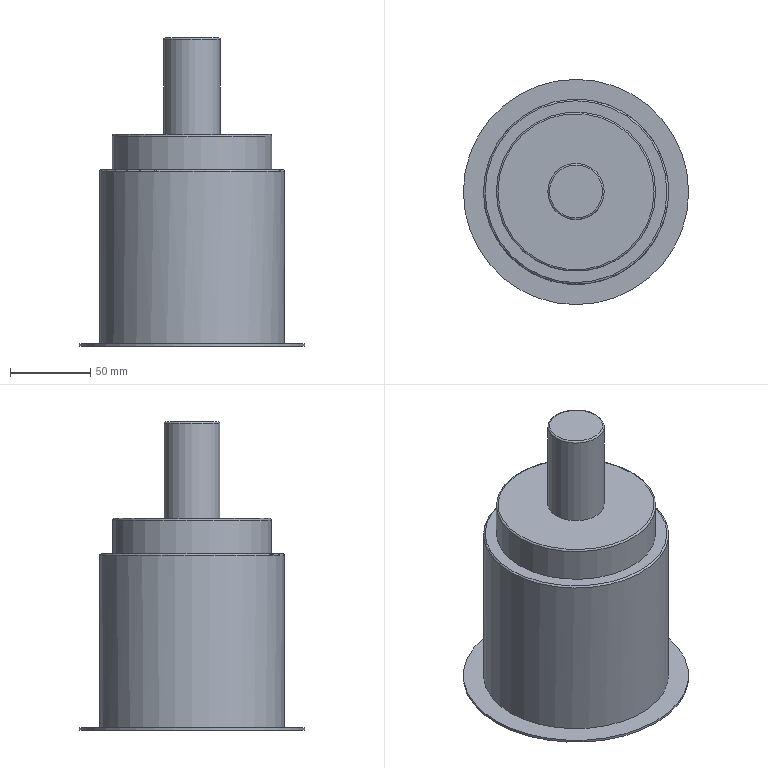Component | NX | A_PART_6 | 1 solid | 12 faces | box 140 x 140 x 191.5 mm | volume 1371784 mm3 | plane 5 | cylinder 4 | torus 3 | commonest cylinder face diameters 99 x1 35 x1 115 x1 140 x1
STEP:
#1=CARTESIAN_POINT('',(0.,0.,0.));
#2=DIRECTION('',(0.,0.,1.));
#3=DIRECTION('',(1.,0.,0.));
#4=AXIS2_PLACEMENT_3D('',#1,#2,#3);
#5=CARTESIAN_POINT('',(303.417,257.136,29.984));
#6=VERTEX_POINT('',#5);
#7=CARTESIAN_POINT('',(352.917,257.26,29.984));
#8=DIRECTION('',(0.,0.,-1.));
#9=DIRECTION('',(-1.,-0.0025,0.));
#10=AXIS2_PLACEMENT_3D('',#7,#8,#9);
#11=CIRCLE('',#10,49.5);
#12=CARTESIAN_POINT('',(352.917,257.26,30.984));
#13=DIRECTION('',(0.,0.,-1.));
#14=DIRECTION('',(-1.,-0.0025,0.));
#15=AXIS2_PLACEMENT_3D('',#12,#13,#14);
#16=CYLINDRICAL_SURFACE('',#15,49.5);
#17=CARTESIAN_POINT('',(0.,1.));
#18=DIRECTION('',(1.,0.));
#19=VECTOR('',#18,1.);
#20=LINE('',#17,#19);
#21=(GEOMETRIC_REPRESENTATION_CONTEXT(2)PARAMETRIC_REPRESENTATION_CONTEXT()REPRESENTATION_CONTEXT('',''));
#22=DEFINITIONAL_REPRESENTATION('',(#20),#21);
#23=PCURVE('',#16,#22);
#24=CARTESIAN_POINT('',(352.917,257.26,29.984));
#25=DIRECTION('',(0.,0.,-1.));
#26=DIRECTION('',(-1.,-0.0025,0.));
#27=AXIS2_PLACEMENT_3D('',#24,#25,#26);
#28=TOROIDAL_SURFACE('',#27,48.5,1.);
#29=CARTESIAN_POINT('',(0.,6.283));
#30=DIRECTION('',(1.,0.));
#31=VECTOR('',#30,1.);
#32=LINE('',#29,#31);
#33=(GEOMETRIC_REPRESENTATION_CONTEXT(2)PARAMETRIC_REPRESENTATION_CONTEXT()REPRESENTATION_CONTEXT('',''));
#34=DEFINITIONAL_REPRESENTATION('',(#32),#33);
#35=PCURVE('',#28,#34);
#36=SURFACE_CURVE('',#11,(#23,#35),.PCURVE_S1.);
#37=EDGE_CURVE('',#6,#6,#36,.T.);
#38=ORIENTED_EDGE('',*,*,#37,.T.);
#39=CARTESIAN_POINT('',(303.417,257.136,8.984));
#40=VERTEX_POINT('',#39);
#41=CARTESIAN_POINT('',(303.417,257.136,29.984));
#42=CARTESIAN_POINT('',(303.417,257.136,8.984));
#43=B_SPLINE_CURVE_WITH_KNOTS('',1,(#41,#42),.UNSPECIFIED.,.F.,.F.,(2,2),(1.,22.),.PIECEWISE_BEZIER_KNOTS.);
#44=CARTESIAN_POINT('',(6.283,0.));
#45=DIRECTION('',(0.,1.));
#46=VECTOR('',#45,1.);
#47=LINE('',#44,#46);
#48=(GEOMETRIC_REPRESENTATION_CONTEXT(2)PARAMETRIC_REPRESENTATION_CONTEXT()REPRESENTATION_CONTEXT('',''));
#49=DEFINITIONAL_REPRESENTATION('',(#47),#48);
#50=PCURVE('',#16,#49);
#51=CARTESIAN_POINT('',(0.,0.));
#52=DIRECTION('',(0.,1.));
#53=VECTOR('',#52,1.);
#54=LINE('',#51,#53);
#55=(GEOMETRIC_REPRESENTATION_CONTEXT(2)PARAMETRIC_REPRESENTATION_CONTEXT()REPRESENTATION_CONTEXT('',''));
#56=DEFINITIONAL_REPRESENTATION('',(#54),#55);
#57=PCURVE('',#16,#56);
#58=SEAM_CURVE('',#43,(#50,#57),.PCURVE_S1.);
#59=EDGE_CURVE('',#6,#40,#58,.T.);
#60=ORIENTED_EDGE('',*,*,#59,.T.);
#61=CARTESIAN_POINT('',(352.917,257.26,8.984));
#62=DIRECTION('',(0.,0.,1.));
#63=DIRECTION('',(-1.,-0.0025,0.));
#64=AXIS2_PLACEMENT_3D('',#61,#62,#63);
#65=CIRCLE('',#64,49.5);
#66=CARTESIAN_POINT('',(6.283,22.));
#67=DIRECTION('',(-1.,0.));
#68=VECTOR('',#67,1.);
#69=LINE('',#66,#68);
#70=(GEOMETRIC_REPRESENTATION_CONTEXT(2)PARAMETRIC_REPRESENTATION_CONTEXT()REPRESENTATION_CONTEXT('',''));
#71=DEFINITIONAL_REPRESENTATION('',(#69),#70);
#72=PCURVE('',#16,#71);
#73=CARTESIAN_POINT('',(352.917,257.26,8.984));
#74=DIRECTION('',(0.,0.,-1.));
#75=DIRECTION('',(-1.,-0.0025,0.));
#76=AXIS2_PLACEMENT_3D('',#73,#74,#75);
#77=PLANE('',#76);
#78=CARTESIAN_POINT('',(49.5,-0.));
#79=CARTESIAN_POINT('',(49.5,-85.737));
#80=CARTESIAN_POINT('',(-24.75,-42.868));
#81=CARTESIAN_POINT('',(-99.,-0.));
#82=CARTESIAN_POINT('',(-24.75,42.868));
#83=CARTESIAN_POINT('',(49.5,85.737));
#84=CARTESIAN_POINT('',(49.5,-0.));
#85=(BOUNDED_CURVE()B_SPLINE_CURVE(2,(#78,#79,#80,#81,#82,#83,#84),.UNSPECIFIED.,.T.,.F.)B_SPLINE_CURVE_WITH_KNOTS((1,2,2,2,2,1),(-2.094,0.,2.094,4.189,6.283,8.378),.UNSPECIFIED.)CURVE()GEOMETRIC_REPRESENTATION_ITEM()RATIONAL_B_SPLINE_CURVE((1.,0.5,1.,0.5,1.,0.5,1.))REPRESENTATION_ITEM(''));
#86=(GEOMETRIC_REPRESENTATION_CONTEXT(2)PARAMETRIC_REPRESENTATION_CONTEXT()REPRESENTATION_CONTEXT('',''));
#87=DEFINITIONAL_REPRESENTATION('',(#85),#86);
#88=PCURVE('',#77,#87);
#89=SURFACE_CURVE('',#65,(#72,#88),.PCURVE_S1.);
#90=EDGE_CURVE('',#40,#40,#89,.T.);
#91=ORIENTED_EDGE('',*,*,#90,.T.);
#92=ORIENTED_EDGE('',*,*,#59,.F.);
#93=EDGE_LOOP('',(#38,#60,#91,#92));
#94=FACE_BOUND('',#93,.T.);
#95=ADVANCED_FACE('',(#94),#16,.T.);
#96=CARTESIAN_POINT('',(304.417,257.138,30.984));
#97=VERTEX_POINT('',#96);
#98=CARTESIAN_POINT('',(352.917,257.26,30.984));
#99=DIRECTION('',(0.,0.,1.));
#100=DIRECTION('',(-1.,-0.0025,0.));
#101=AXIS2_PLACEMENT_3D('',#98,#99,#100);
#102=CIRCLE('',#101,48.5);
#103=CARTESIAN_POINT('',(352.917,257.26,30.984));
#104=DIRECTION('',(0.,0.,-1.));
#105=DIRECTION('',(-1.,-0.0025,0.));
#106=AXIS2_PLACEMENT_3D('',#103,#104,#105);
#107=PLANE('',#106);
#108=CARTESIAN_POINT('',(48.5,-0.));
#109=CARTESIAN_POINT('',(48.5,-84.004));
#110=CARTESIAN_POINT('',(-24.25,-42.002));
#111=CARTESIAN_POINT('',(-97.,0.));
#112=CARTESIAN_POINT('',(-24.25,42.002));
#113=CARTESIAN_POINT('',(48.5,84.004));
#114=CARTESIAN_POINT('',(48.5,-0.));
#115=(BOUNDED_CURVE()B_SPLINE_CURVE(2,(#108,#109,#110,#111,#112,#113,#114),.UNSPECIFIED.,.T.,.F.)B_SPLINE_CURVE_WITH_KNOTS((1,2,2,2,2,1),(-2.094,0.,2.094,4.189,6.283,8.378),.UNSPECIFIED.)CURVE()GEOMETRIC_REPRESENTATION_ITEM()RATIONAL_B_SPLINE_CURVE((1.,0.5,1.,0.5,1.,0.5,1.))REPRESENTATION_ITEM(''));
#116=(GEOMETRIC_REPRESENTATION_CONTEXT(2)PARAMETRIC_REPRESENTATION_CONTEXT()REPRESENTATION_CONTEXT('',''));
#117=DEFINITIONAL_REPRESENTATION('',(#115),#116);
#118=PCURVE('',#107,#117);
#119=CARTESIAN_POINT('',(6.283,4.712));
#120=DIRECTION('',(-1.,0.));
#121=VECTOR('',#120,1.);
#122=LINE('',#119,#121);
#123=(GEOMETRIC_REPRESENTATION_CONTEXT(2)PARAMETRIC_REPRESENTATION_CONTEXT()REPRESENTATION_CONTEXT('',''));
#124=DEFINITIONAL_REPRESENTATION('',(#122),#123);
#125=PCURVE('',#28,#124);
#126=SURFACE_CURVE('',#102,(#118,#125),.PCURVE_S1.);
#127=EDGE_CURVE('',#97,#97,#126,.T.);
#128=ORIENTED_EDGE('',*,*,#127,.T.);
#129=EDGE_LOOP('',(#128));
#130=FACE_BOUND('',#129,.T.);
#131=CARTESIAN_POINT('',(370.417,257.303,30.984));
#132=VERTEX_POINT('',#131);
#133=CARTESIAN_POINT('',(335.417,257.216,30.984));
#134=VERTEX_POINT('',#133);
#135=CARTESIAN_POINT('',(352.917,257.26,30.984));
#136=DIRECTION('',(0.,0.,-1.));
#137=DIRECTION('',(1.,0.0025,0.));
#138=AXIS2_PLACEMENT_3D('',#135,#136,#137);
#139=CIRCLE('',#138,17.5);
#140=CARTESIAN_POINT('',(0.,0.));
#141=DIRECTION('',(-1.,0.));
#142=AXIS2_PLACEMENT_2D('',#140,#141);
#143=CIRCLE('',#142,17.5);
#144=(GEOMETRIC_REPRESENTATION_CONTEXT(2)PARAMETRIC_REPRESENTATION_CONTEXT()REPRESENTATION_CONTEXT('',''));
#145=DEFINITIONAL_REPRESENTATION('',(#143),#144);
#146=PCURVE('',#107,#145);
#147=CARTESIAN_POINT('',(352.917,257.26,90.984));
#148=DIRECTION('',(0.,0.,-1.));
#149=DIRECTION('',(-1.,-0.0025,0.));
#150=AXIS2_PLACEMENT_3D('',#147,#148,#149);
#151=CYLINDRICAL_SURFACE('',#150,17.5);
#152=CARTESIAN_POINT('',(3.142,60.));
#153=DIRECTION('',(1.,0.));
#154=VECTOR('',#153,1.);
#155=LINE('',#152,#154);
#156=(GEOMETRIC_REPRESENTATION_CONTEXT(2)PARAMETRIC_REPRESENTATION_CONTEXT()REPRESENTATION_CONTEXT('',''));
#157=DEFINITIONAL_REPRESENTATION('',(#155),#156);
#158=PCURVE('',#151,#157);
#159=SURFACE_CURVE('',#139,(#146,#158),.PCURVE_S1.);
#160=EDGE_CURVE('',#132,#134,#159,.T.);
#161=ORIENTED_EDGE('',*,*,#160,.T.);
#162=CARTESIAN_POINT('',(352.917,257.26,30.984));
#163=DIRECTION('',(0.,0.,-1.));
#164=DIRECTION('',(1.,0.0025,0.));
#165=AXIS2_PLACEMENT_3D('',#162,#163,#164);
#166=CIRCLE('',#165,17.5);
#167=CARTESIAN_POINT('',(0.,0.));
#168=DIRECTION('',(-1.,0.));
#169=AXIS2_PLACEMENT_2D('',#167,#168);
#170=CIRCLE('',#169,17.5);
#171=(GEOMETRIC_REPRESENTATION_CONTEXT(2)PARAMETRIC_REPRESENTATION_CONTEXT()REPRESENTATION_CONTEXT('',''));
#172=DEFINITIONAL_REPRESENTATION('',(#170),#171);
#173=PCURVE('',#107,#172);
#174=CARTESIAN_POINT('',(-3.142,60.));
#175=DIRECTION('',(1.,0.));
#176=VECTOR('',#175,1.);
#177=LINE('',#174,#176);
#178=(GEOMETRIC_REPRESENTATION_CONTEXT(2)PARAMETRIC_REPRESENTATION_CONTEXT()REPRESENTATION_CONTEXT('',''));
#179=DEFINITIONAL_REPRESENTATION('',(#177),#178);
#180=PCURVE('',#151,#179);
#181=SURFACE_CURVE('',#166,(#173,#180),.PCURVE_S1.);
#182=EDGE_CURVE('',#134,#132,#181,.T.);
#183=ORIENTED_EDGE('',*,*,#182,.T.);
#184=EDGE_LOOP('',(#161,#183));
#185=FACE_BOUND('',#184,.T.);
#186=ADVANCED_FACE('',(#130,#185),#107,.F.);
#187=CARTESIAN_POINT('',(335.417,257.216,89.984));
#188=VERTEX_POINT('',#187);
#189=CARTESIAN_POINT('',(352.917,257.26,89.984));
#190=DIRECTION('',(0.,0.,-1.));
#191=DIRECTION('',(-1.,-0.0025,0.));
#192=AXIS2_PLACEMENT_3D('',#189,#190,#191);
#193=CIRCLE('',#192,17.5);
#194=CARTESIAN_POINT('',(0.,1.));
#195=DIRECTION('',(1.,0.));
#196=VECTOR('',#195,1.);
#197=LINE('',#194,#196);
#198=(GEOMETRIC_REPRESENTATION_CONTEXT(2)PARAMETRIC_REPRESENTATION_CONTEXT()REPRESENTATION_CONTEXT('',''));
#199=DEFINITIONAL_REPRESENTATION('',(#197),#198);
#200=PCURVE('',#151,#199);
#201=CARTESIAN_POINT('',(352.917,257.26,89.984));
#202=DIRECTION('',(0.,0.,-1.));
#203=DIRECTION('',(-1.,-0.0025,0.));
#204=AXIS2_PLACEMENT_3D('',#201,#202,#203);
#205=TOROIDAL_SURFACE('',#204,16.5,1.);
#206=CARTESIAN_POINT('',(0.,6.283));
#207=DIRECTION('',(1.,0.));
#208=VECTOR('',#207,1.);
#209=LINE('',#206,#208);
#210=(GEOMETRIC_REPRESENTATION_CONTEXT(2)PARAMETRIC_REPRESENTATION_CONTEXT()REPRESENTATION_CONTEXT('',''));
#211=DEFINITIONAL_REPRESENTATION('',(#209),#210);
#212=PCURVE('',#205,#211);
#213=SURFACE_CURVE('',#193,(#200,#212),.PCURVE_S1.);
#214=EDGE_CURVE('',#188,#188,#213,.T.);
#215=ORIENTED_EDGE('',*,*,#214,.T.);
#216=CARTESIAN_POINT('',(335.417,257.216,89.984));
#217=CARTESIAN_POINT('',(335.417,257.216,30.984));
#218=B_SPLINE_CURVE_WITH_KNOTS('',1,(#216,#217),.UNSPECIFIED.,.F.,.F.,(2,2),(1.,60.),.PIECEWISE_BEZIER_KNOTS.);
#219=CARTESIAN_POINT('',(6.283,0.));
#220=DIRECTION('',(0.,1.));
#221=VECTOR('',#220,1.);
#222=LINE('',#219,#221);
#223=(GEOMETRIC_REPRESENTATION_CONTEXT(2)PARAMETRIC_REPRESENTATION_CONTEXT()REPRESENTATION_CONTEXT('',''));
#224=DEFINITIONAL_REPRESENTATION('',(#222),#223);
#225=PCURVE('',#151,#224);
#226=CARTESIAN_POINT('',(0.,0.));
#227=DIRECTION('',(0.,1.));
#228=VECTOR('',#227,1.);
#229=LINE('',#226,#228);
#230=(GEOMETRIC_REPRESENTATION_CONTEXT(2)PARAMETRIC_REPRESENTATION_CONTEXT()REPRESENTATION_CONTEXT('',''));
#231=DEFINITIONAL_REPRESENTATION('',(#229),#230);
#232=PCURVE('',#151,#231);
#233=SEAM_CURVE('',#218,(#225,#232),.PCURVE_S1.);
#234=EDGE_CURVE('',#188,#134,#233,.T.);
#235=ORIENTED_EDGE('',*,*,#234,.T.);
#236=ORIENTED_EDGE('',*,*,#160,.F.);
#237=ORIENTED_EDGE('',*,*,#182,.F.);
#238=ORIENTED_EDGE('',*,*,#234,.F.);
#239=EDGE_LOOP('',(#215,#235,#236,#237,#238));
#240=FACE_BOUND('',#239,.T.);
#241=ADVANCED_FACE('',(#240),#151,.T.);
#242=CARTESIAN_POINT('',(336.417,257.218,90.984));
#243=VERTEX_POINT('',#242);
#244=CARTESIAN_POINT('',(352.917,257.26,90.984));
#245=DIRECTION('',(0.,0.,1.));
#246=DIRECTION('',(-1.,-0.0025,0.));
#247=AXIS2_PLACEMENT_3D('',#244,#245,#246);
#248=CIRCLE('',#247,16.5);
#249=CARTESIAN_POINT('',(352.917,257.26,90.984));
#250=DIRECTION('',(0.,0.,-1.));
#251=DIRECTION('',(-1.,-0.0025,0.));
#252=AXIS2_PLACEMENT_3D('',#249,#250,#251);
#253=PLANE('',#252);
#254=CARTESIAN_POINT('',(16.5,0.));
#255=CARTESIAN_POINT('',(16.5,-28.579));
#256=CARTESIAN_POINT('',(-8.25,-14.289));
#257=CARTESIAN_POINT('',(-33.,-0.));
#258=CARTESIAN_POINT('',(-8.25,14.289));
#259=CARTESIAN_POINT('',(16.5,28.579));
#260=CARTESIAN_POINT('',(16.5,0.));
#261=(BOUNDED_CURVE()B_SPLINE_CURVE(2,(#254,#255,#256,#257,#258,#259,#260),.UNSPECIFIED.,.T.,.F.)B_SPLINE_CURVE_WITH_KNOTS((1,2,2,2,2,1),(-2.094,0.,2.094,4.189,6.283,8.378),.UNSPECIFIED.)CURVE()GEOMETRIC_REPRESENTATION_ITEM()RATIONAL_B_SPLINE_CURVE((1.,0.5,1.,0.5,1.,0.5,1.))REPRESENTATION_ITEM(''));
#262=(GEOMETRIC_REPRESENTATION_CONTEXT(2)PARAMETRIC_REPRESENTATION_CONTEXT()REPRESENTATION_CONTEXT('',''));
#263=DEFINITIONAL_REPRESENTATION('',(#261),#262);
#264=PCURVE('',#253,#263);
#265=CARTESIAN_POINT('',(6.283,4.712));
#266=DIRECTION('',(-1.,0.));
#267=VECTOR('',#266,1.);
#268=LINE('',#265,#267);
#269=(GEOMETRIC_REPRESENTATION_CONTEXT(2)PARAMETRIC_REPRESENTATION_CONTEXT()REPRESENTATION_CONTEXT('',''));
#270=DEFINITIONAL_REPRESENTATION('',(#268),#269);
#271=PCURVE('',#205,#270);
#272=SURFACE_CURVE('',#248,(#264,#271),.PCURVE_S1.);
#273=EDGE_CURVE('',#243,#243,#272,.T.);
#274=ORIENTED_EDGE('',*,*,#273,.T.);
#275=EDGE_LOOP('',(#274));
#276=FACE_BOUND('',#275,.T.);
#277=ADVANCED_FACE('',(#276),#253,.F.);
#278=ORIENTED_EDGE('',*,*,#273,.F.);
#279=CARTESIAN_POINT('',(336.417,257.218,90.984));
#280=CARTESIAN_POINT('',(336.15,257.218,90.984));
#281=CARTESIAN_POINT('',(335.889,257.217,90.899));
#282=CARTESIAN_POINT('',(335.665,257.216,90.736));
#283=CARTESIAN_POINT('',(335.502,257.216,90.511));
#284=CARTESIAN_POINT('',(335.417,257.216,90.251));
#285=CARTESIAN_POINT('',(335.417,257.216,89.984));
#286=(BOUNDED_CURVE()B_SPLINE_CURVE(6,(#279,#280,#281,#282,#283,#284,#285),.UNSPECIFIED.,.F.,.F.)B_SPLINE_CURVE_WITH_KNOTS((7,7),(4.712,6.283),.PIECEWISE_BEZIER_KNOTS.)CURVE()GEOMETRIC_REPRESENTATION_ITEM()RATIONAL_B_SPLINE_CURVE((1.031,1.01,0.9979,0.994,0.9979,1.01,1.031))REPRESENTATION_ITEM(''));
#287=CARTESIAN_POINT('',(6.283,0.));
#288=DIRECTION('',(0.,1.));
#289=VECTOR('',#288,1.);
#290=LINE('',#287,#289);
#291=(GEOMETRIC_REPRESENTATION_CONTEXT(2)PARAMETRIC_REPRESENTATION_CONTEXT()REPRESENTATION_CONTEXT('',''));
#292=DEFINITIONAL_REPRESENTATION('',(#290),#291);
#293=PCURVE('',#205,#292);
#294=CARTESIAN_POINT('',(0.,0.));
#295=DIRECTION('',(0.,1.));
#296=VECTOR('',#295,1.);
#297=LINE('',#294,#296);
#298=(GEOMETRIC_REPRESENTATION_CONTEXT(2)PARAMETRIC_REPRESENTATION_CONTEXT()REPRESENTATION_CONTEXT('',''));
#299=DEFINITIONAL_REPRESENTATION('',(#297),#298);
#300=PCURVE('',#205,#299);
#301=SEAM_CURVE('',#286,(#293,#300),.PCURVE_S1.);
#302=EDGE_CURVE('',#243,#188,#301,.T.);
#303=ORIENTED_EDGE('',*,*,#302,.T.);
#304=ORIENTED_EDGE('',*,*,#214,.F.);
#305=ORIENTED_EDGE('',*,*,#302,.F.);
#306=EDGE_LOOP('',(#278,#303,#304,#305));
#307=FACE_BOUND('',#306,.T.);
#308=ADVANCED_FACE('',(#307),#205,.T.);
#309=ORIENTED_EDGE('',*,*,#127,.F.);
#310=CARTESIAN_POINT('',(304.417,257.138,30.984));
#311=CARTESIAN_POINT('',(304.15,257.138,30.984));
#312=CARTESIAN_POINT('',(303.889,257.137,30.899));
#313=CARTESIAN_POINT('',(303.665,257.136,30.736));
#314=CARTESIAN_POINT('',(303.502,257.136,30.511));
#315=CARTESIAN_POINT('',(303.417,257.136,30.251));
#316=CARTESIAN_POINT('',(303.417,257.136,29.984));
#317=(BOUNDED_CURVE()B_SPLINE_CURVE(6,(#310,#311,#312,#313,#314,#315,#316),.UNSPECIFIED.,.F.,.F.)B_SPLINE_CURVE_WITH_KNOTS((7,7),(4.712,6.283),.PIECEWISE_BEZIER_KNOTS.)CURVE()GEOMETRIC_REPRESENTATION_ITEM()RATIONAL_B_SPLINE_CURVE((1.031,1.01,0.9979,0.994,0.9979,1.01,1.031))REPRESENTATION_ITEM(''));
#318=CARTESIAN_POINT('',(6.283,0.));
#319=DIRECTION('',(0.,1.));
#320=VECTOR('',#319,1.);
#321=LINE('',#318,#320);
#322=(GEOMETRIC_REPRESENTATION_CONTEXT(2)PARAMETRIC_REPRESENTATION_CONTEXT()REPRESENTATION_CONTEXT('',''));
#323=DEFINITIONAL_REPRESENTATION('',(#321),#322);
#324=PCURVE('',#28,#323);
#325=CARTESIAN_POINT('',(0.,0.));
#326=DIRECTION('',(0.,1.));
#327=VECTOR('',#326,1.);
#328=LINE('',#325,#327);
#329=(GEOMETRIC_REPRESENTATION_CONTEXT(2)PARAMETRIC_REPRESENTATION_CONTEXT()REPRESENTATION_CONTEXT('',''));
#330=DEFINITIONAL_REPRESENTATION('',(#328),#329);
#331=PCURVE('',#28,#330);
#332=SEAM_CURVE('',#317,(#324,#331),.PCURVE_S1.);
#333=EDGE_CURVE('',#97,#6,#332,.T.);
#334=ORIENTED_EDGE('',*,*,#333,.T.);
#335=ORIENTED_EDGE('',*,*,#37,.F.);
#336=ORIENTED_EDGE('',*,*,#333,.F.);
#337=EDGE_LOOP('',(#309,#334,#335,#336));
#338=FACE_BOUND('',#337,.T.);
#339=ADVANCED_FACE('',(#338),#28,.T.);
#340=CARTESIAN_POINT('',(295.417,257.116,7.984));
#341=VERTEX_POINT('',#340);
#342=CARTESIAN_POINT('',(352.917,257.26,7.984));
#343=DIRECTION('',(0.,0.,-1.));
#344=DIRECTION('',(-1.,-0.0025,0.));
#345=AXIS2_PLACEMENT_3D('',#342,#343,#344);
#346=CIRCLE('',#345,57.5);
#347=CARTESIAN_POINT('',(352.917,257.26,8.984));
#348=DIRECTION('',(0.,0.,-1.));
#349=DIRECTION('',(-1.,-0.0025,0.));
#350=AXIS2_PLACEMENT_3D('',#347,#348,#349);
#351=CYLINDRICAL_SURFACE('',#350,57.5);
#352=CARTESIAN_POINT('',(0.,1.));
#353=DIRECTION('',(1.,0.));
#354=VECTOR('',#353,1.);
#355=LINE('',#352,#354);
#356=(GEOMETRIC_REPRESENTATION_CONTEXT(2)PARAMETRIC_REPRESENTATION_CONTEXT()REPRESENTATION_CONTEXT('',''));
#357=DEFINITIONAL_REPRESENTATION('',(#355),#356);
#358=PCURVE('',#351,#357);
#359=CARTESIAN_POINT('',(352.917,257.26,7.984));
#360=DIRECTION('',(0.,0.,-1.));
#361=DIRECTION('',(-1.,-0.0025,0.));
#362=AXIS2_PLACEMENT_3D('',#359,#360,#361);
#363=TOROIDAL_SURFACE('',#362,56.5,1.);
#364=CARTESIAN_POINT('',(0.,6.283));
#365=DIRECTION('',(1.,0.));
#366=VECTOR('',#365,1.);
#367=LINE('',#364,#366);
#368=(GEOMETRIC_REPRESENTATION_CONTEXT(2)PARAMETRIC_REPRESENTATION_CONTEXT()REPRESENTATION_CONTEXT('',''));
#369=DEFINITIONAL_REPRESENTATION('',(#367),#368);
#370=PCURVE('',#363,#369);
#371=SURFACE_CURVE('',#346,(#358,#370),.PCURVE_S1.);
#372=EDGE_CURVE('',#341,#341,#371,.T.);
#373=ORIENTED_EDGE('',*,*,#372,.T.);
#374=CARTESIAN_POINT('',(295.417,257.116,-99.016));
#375=VERTEX_POINT('',#374);
#376=CARTESIAN_POINT('',(295.417,257.116,7.984));
#377=CARTESIAN_POINT('',(295.417,257.116,-99.016));
#378=B_SPLINE_CURVE_WITH_KNOTS('',1,(#376,#377),.UNSPECIFIED.,.F.,.F.,(2,2),(1.,108.),.PIECEWISE_BEZIER_KNOTS.);
#379=CARTESIAN_POINT('',(6.283,0.));
#380=DIRECTION('',(0.,1.));
#381=VECTOR('',#380,1.);
#382=LINE('',#379,#381);
#383=(GEOMETRIC_REPRESENTATION_CONTEXT(2)PARAMETRIC_REPRESENTATION_CONTEXT()REPRESENTATION_CONTEXT('',''));
#384=DEFINITIONAL_REPRESENTATION('',(#382),#383);
#385=PCURVE('',#351,#384);
#386=CARTESIAN_POINT('',(0.,0.));
#387=DIRECTION('',(0.,1.));
#388=VECTOR('',#387,1.);
#389=LINE('',#386,#388);
#390=(GEOMETRIC_REPRESENTATION_CONTEXT(2)PARAMETRIC_REPRESENTATION_CONTEXT()REPRESENTATION_CONTEXT('',''));
#391=DEFINITIONAL_REPRESENTATION('',(#389),#390);
#392=PCURVE('',#351,#391);
#393=SEAM_CURVE('',#378,(#385,#392),.PCURVE_S1.);
#394=EDGE_CURVE('',#341,#375,#393,.T.);
#395=ORIENTED_EDGE('',*,*,#394,.T.);
#396=CARTESIAN_POINT('',(410.417,257.403,-99.016));
#397=VERTEX_POINT('',#396);
#398=CARTESIAN_POINT('',(352.917,257.26,-99.016));
#399=DIRECTION('',(0.,0.,-1.));
#400=DIRECTION('',(1.,0.0025,0.));
#401=AXIS2_PLACEMENT_3D('',#398,#399,#400);
#402=CIRCLE('',#401,57.5);
#403=CARTESIAN_POINT('',(3.142,108.));
#404=DIRECTION('',(1.,0.));
#405=VECTOR('',#404,1.);
#406=LINE('',#403,#405);
#407=(GEOMETRIC_REPRESENTATION_CONTEXT(2)PARAMETRIC_REPRESENTATION_CONTEXT()REPRESENTATION_CONTEXT('',''));
#408=DEFINITIONAL_REPRESENTATION('',(#406),#407);
#409=PCURVE('',#351,#408);
#410=CARTESIAN_POINT('',(352.917,257.26,-99.016));
#411=DIRECTION('',(0.,0.,1.));
#412=DIRECTION('',(1.,0.0025,0.));
#413=AXIS2_PLACEMENT_3D('',#410,#411,#412);
#414=PLANE('',#413);
#415=CARTESIAN_POINT('',(57.5,0.));
#416=CARTESIAN_POINT('',(57.5,-99.593));
#417=CARTESIAN_POINT('',(-28.75,-49.796));
#418=CARTESIAN_POINT('',(-115.,-0.));
#419=CARTESIAN_POINT('',(-28.75,49.796));
#420=CARTESIAN_POINT('',(57.5,99.593));
#421=CARTESIAN_POINT('',(57.5,0.));
#422=(BOUNDED_CURVE()B_SPLINE_CURVE(2,(#415,#416,#417,#418,#419,#420,#421),.UNSPECIFIED.,.T.,.F.)B_SPLINE_CURVE_WITH_KNOTS((1,2,2,2,2,1),(-2.094,0.,2.094,4.189,6.283,8.378),.UNSPECIFIED.)CURVE()GEOMETRIC_REPRESENTATION_ITEM()RATIONAL_B_SPLINE_CURVE((1.,0.5,1.,0.5,1.,0.5,1.))REPRESENTATION_ITEM(''));
#423=(GEOMETRIC_REPRESENTATION_CONTEXT(2)PARAMETRIC_REPRESENTATION_CONTEXT()REPRESENTATION_CONTEXT('',''));
#424=DEFINITIONAL_REPRESENTATION('',(#422),#423);
#425=PCURVE('',#414,#424);
#426=SURFACE_CURVE('',#402,(#409,#425),.PCURVE_S1.);
#427=EDGE_CURVE('',#397,#375,#426,.T.);
#428=ORIENTED_EDGE('',*,*,#427,.F.);
#429=CARTESIAN_POINT('',(352.917,257.26,-99.016));
#430=DIRECTION('',(0.,0.,-1.));
#431=DIRECTION('',(1.,0.0025,0.));
#432=AXIS2_PLACEMENT_3D('',#429,#430,#431);
#433=CIRCLE('',#432,57.5);
#434=CARTESIAN_POINT('',(-3.142,108.));
#435=DIRECTION('',(1.,0.));
#436=VECTOR('',#435,1.);
#437=LINE('',#434,#436);
#438=(GEOMETRIC_REPRESENTATION_CONTEXT(2)PARAMETRIC_REPRESENTATION_CONTEXT()REPRESENTATION_CONTEXT('',''));
#439=DEFINITIONAL_REPRESENTATION('',(#437),#438);
#440=PCURVE('',#351,#439);
#441=CARTESIAN_POINT('',(57.5,0.));
#442=CARTESIAN_POINT('',(57.5,-99.593));
#443=CARTESIAN_POINT('',(-28.75,-49.796));
#444=CARTESIAN_POINT('',(-115.,-0.));
#445=CARTESIAN_POINT('',(-28.75,49.796));
#446=CARTESIAN_POINT('',(57.5,99.593));
#447=CARTESIAN_POINT('',(57.5,0.));
#448=(BOUNDED_CURVE()B_SPLINE_CURVE(2,(#441,#442,#443,#444,#445,#446,#447),.UNSPECIFIED.,.T.,.F.)B_SPLINE_CURVE_WITH_KNOTS((1,2,2,2,2,1),(-2.094,0.,2.094,4.189,6.283,8.378),.UNSPECIFIED.)CURVE()GEOMETRIC_REPRESENTATION_ITEM()RATIONAL_B_SPLINE_CURVE((1.,0.5,1.,0.5,1.,0.5,1.))REPRESENTATION_ITEM(''));
#449=(GEOMETRIC_REPRESENTATION_CONTEXT(2)PARAMETRIC_REPRESENTATION_CONTEXT()REPRESENTATION_CONTEXT('',''));
#450=DEFINITIONAL_REPRESENTATION('',(#448),#449);
#451=PCURVE('',#414,#450);
#452=SURFACE_CURVE('',#433,(#440,#451),.PCURVE_S1.);
#453=EDGE_CURVE('',#375,#397,#452,.T.);
#454=ORIENTED_EDGE('',*,*,#453,.F.);
#455=ORIENTED_EDGE('',*,*,#394,.F.);
#456=EDGE_LOOP('',(#373,#395,#428,#454,#455));
#457=FACE_BOUND('',#456,.T.);
#458=ADVANCED_FACE('',(#457),#351,.T.);
#459=CARTESIAN_POINT('',(296.417,257.118,8.984));
#460=VERTEX_POINT('',#459);
#461=CARTESIAN_POINT('',(352.917,257.26,8.984));
#462=DIRECTION('',(0.,0.,1.));
#463=DIRECTION('',(-1.,-0.0025,0.));
#464=AXIS2_PLACEMENT_3D('',#461,#462,#463);
#465=CIRCLE('',#464,56.5);
#466=CARTESIAN_POINT('',(56.5,0.));
#467=CARTESIAN_POINT('',(56.5,-97.861));
#468=CARTESIAN_POINT('',(-28.25,-48.93));
#469=CARTESIAN_POINT('',(-113.,-0.));
#470=CARTESIAN_POINT('',(-28.25,48.93));
#471=CARTESIAN_POINT('',(56.5,97.861));
#472=CARTESIAN_POINT('',(56.5,0.));
#473=(BOUNDED_CURVE()B_SPLINE_CURVE(2,(#466,#467,#468,#469,#470,#471,#472),.UNSPECIFIED.,.T.,.F.)B_SPLINE_CURVE_WITH_KNOTS((1,2,2,2,2,1),(-2.094,0.,2.094,4.189,6.283,8.378),.UNSPECIFIED.)CURVE()GEOMETRIC_REPRESENTATION_ITEM()RATIONAL_B_SPLINE_CURVE((1.,0.5,1.,0.5,1.,0.5,1.))REPRESENTATION_ITEM(''));
#474=(GEOMETRIC_REPRESENTATION_CONTEXT(2)PARAMETRIC_REPRESENTATION_CONTEXT()REPRESENTATION_CONTEXT('',''));
#475=DEFINITIONAL_REPRESENTATION('',(#473),#474);
#476=PCURVE('',#77,#475);
#477=CARTESIAN_POINT('',(6.283,4.712));
#478=DIRECTION('',(-1.,0.));
#479=VECTOR('',#478,1.);
#480=LINE('',#477,#479);
#481=(GEOMETRIC_REPRESENTATION_CONTEXT(2)PARAMETRIC_REPRESENTATION_CONTEXT()REPRESENTATION_CONTEXT('',''));
#482=DEFINITIONAL_REPRESENTATION('',(#480),#481);
#483=PCURVE('',#363,#482);
#484=SURFACE_CURVE('',#465,(#476,#483),.PCURVE_S1.);
#485=EDGE_CURVE('',#460,#460,#484,.T.);
#486=ORIENTED_EDGE('',*,*,#485,.T.);
#487=EDGE_LOOP('',(#486));
#488=FACE_BOUND('',#487,.T.);
#489=ORIENTED_EDGE('',*,*,#90,.F.);
#490=EDGE_LOOP('',(#489));
#491=FACE_BOUND('',#490,.T.);
#492=ADVANCED_FACE('',(#488,#491),#77,.F.);
#493=ORIENTED_EDGE('',*,*,#485,.F.);
#494=CARTESIAN_POINT('',(296.417,257.118,8.984));
#495=CARTESIAN_POINT('',(296.15,257.118,8.984));
#496=CARTESIAN_POINT('',(295.889,257.117,8.899));
#497=CARTESIAN_POINT('',(295.665,257.116,8.736));
#498=CARTESIAN_POINT('',(295.502,257.116,8.511));
#499=CARTESIAN_POINT('',(295.417,257.116,8.251));
#500=CARTESIAN_POINT('',(295.417,257.116,7.984));
#501=(BOUNDED_CURVE()B_SPLINE_CURVE(6,(#494,#495,#496,#497,#498,#499,#500),.UNSPECIFIED.,.F.,.F.)B_SPLINE_CURVE_WITH_KNOTS((7,7),(4.712,6.283),.PIECEWISE_BEZIER_KNOTS.)CURVE()GEOMETRIC_REPRESENTATION_ITEM()RATIONAL_B_SPLINE_CURVE((1.031,1.01,0.9979,0.994,0.9979,1.01,1.031))REPRESENTATION_ITEM(''));
#502=CARTESIAN_POINT('',(6.283,0.));
#503=DIRECTION('',(0.,1.));
#504=VECTOR('',#503,1.);
#505=LINE('',#502,#504);
#506=(GEOMETRIC_REPRESENTATION_CONTEXT(2)PARAMETRIC_REPRESENTATION_CONTEXT()REPRESENTATION_CONTEXT('',''));
#507=DEFINITIONAL_REPRESENTATION('',(#505),#506);
#508=PCURVE('',#363,#507);
#509=CARTESIAN_POINT('',(0.,0.));
#510=DIRECTION('',(0.,1.));
#511=VECTOR('',#510,1.);
#512=LINE('',#509,#511);
#513=(GEOMETRIC_REPRESENTATION_CONTEXT(2)PARAMETRIC_REPRESENTATION_CONTEXT()REPRESENTATION_CONTEXT('',''));
#514=DEFINITIONAL_REPRESENTATION('',(#512),#513);
#515=PCURVE('',#363,#514);
#516=SEAM_CURVE('',#501,(#508,#515),.PCURVE_S1.);
#517=EDGE_CURVE('',#460,#341,#516,.T.);
#518=ORIENTED_EDGE('',*,*,#517,.T.);
#519=ORIENTED_EDGE('',*,*,#372,.F.);
#520=ORIENTED_EDGE('',*,*,#517,.F.);
#521=EDGE_LOOP('',(#493,#518,#519,#520));
#522=FACE_BOUND('',#521,.T.);
#523=ADVANCED_FACE('',(#522),#363,.T.);
#524=CARTESIAN_POINT('',(422.917,257.435,-100.516));
#525=VERTEX_POINT('',#524);
#526=CARTESIAN_POINT('',(352.917,257.26,-100.516));
#527=DIRECTION('',(0.,0.,1.));
#528=DIRECTION('',(1.,0.0025,0.));
#529=AXIS2_PLACEMENT_3D('',#526,#527,#528);
#530=CIRCLE('',#529,70.);
#531=CARTESIAN_POINT('',(352.917,257.26,-100.516));
#532=DIRECTION('',(0.,0.,1.));
#533=DIRECTION('',(1.,0.0025,0.));
#534=AXIS2_PLACEMENT_3D('',#531,#532,#533);
#535=CYLINDRICAL_SURFACE('',#534,70.);
#536=CARTESIAN_POINT('',(0.,0.));
#537=DIRECTION('',(1.,0.));
#538=VECTOR('',#537,1.);
#539=LINE('',#536,#538);
#540=(GEOMETRIC_REPRESENTATION_CONTEXT(2)PARAMETRIC_REPRESENTATION_CONTEXT()REPRESENTATION_CONTEXT('',''));
#541=DEFINITIONAL_REPRESENTATION('',(#539),#540);
#542=PCURVE('',#535,#541);
#543=CARTESIAN_POINT('',(352.917,257.26,-100.516));
#544=DIRECTION('',(0.,0.,1.));
#545=DIRECTION('',(1.,0.0025,0.));
#546=AXIS2_PLACEMENT_3D('',#543,#544,#545);
#547=PLANE('',#546);
#548=CARTESIAN_POINT('',(0.,0.));
#549=DIRECTION('',(1.,0.));
#550=AXIS2_PLACEMENT_2D('',#548,#549);
#551=CIRCLE('',#550,70.);
#552=(GEOMETRIC_REPRESENTATION_CONTEXT(2)PARAMETRIC_REPRESENTATION_CONTEXT()REPRESENTATION_CONTEXT('',''));
#553=DEFINITIONAL_REPRESENTATION('',(#551),#552);
#554=PCURVE('',#547,#553);
#555=SURFACE_CURVE('',#530,(#542,#554),.PCURVE_S1.);
#556=EDGE_CURVE('',#525,#525,#555,.T.);
#557=ORIENTED_EDGE('',*,*,#556,.T.);
#558=CARTESIAN_POINT('',(422.917,257.435,-99.016));
#559=VERTEX_POINT('',#558);
#560=CARTESIAN_POINT('',(422.917,257.435,-100.516));
#561=CARTESIAN_POINT('',(422.917,257.435,-99.016));
#562=B_SPLINE_CURVE_WITH_KNOTS('',1,(#560,#561),.UNSPECIFIED.,.F.,.F.,(2,2),(0.,1.5),.PIECEWISE_BEZIER_KNOTS.);
#563=CARTESIAN_POINT('',(6.283,0.));
#564=DIRECTION('',(0.,1.));
#565=VECTOR('',#564,1.);
#566=LINE('',#563,#565);
#567=(GEOMETRIC_REPRESENTATION_CONTEXT(2)PARAMETRIC_REPRESENTATION_CONTEXT()REPRESENTATION_CONTEXT('',''));
#568=DEFINITIONAL_REPRESENTATION('',(#566),#567);
#569=PCURVE('',#535,#568);
#570=CARTESIAN_POINT('',(0.,0.));
#571=DIRECTION('',(0.,1.));
#572=VECTOR('',#571,1.);
#573=LINE('',#570,#572);
#574=(GEOMETRIC_REPRESENTATION_CONTEXT(2)PARAMETRIC_REPRESENTATION_CONTEXT()REPRESENTATION_CONTEXT('',''));
#575=DEFINITIONAL_REPRESENTATION('',(#573),#574);
#576=PCURVE('',#535,#575);
#577=SEAM_CURVE('',#562,(#569,#576),.PCURVE_S1.);
#578=EDGE_CURVE('',#525,#559,#577,.T.);
#579=ORIENTED_EDGE('',*,*,#578,.T.);
#580=CARTESIAN_POINT('',(352.917,257.26,-99.016));
#581=DIRECTION('',(0.,0.,1.));
#582=DIRECTION('',(1.,0.0025,0.));
#583=AXIS2_PLACEMENT_3D('',#580,#581,#582);
#584=CIRCLE('',#583,70.);
#585=CARTESIAN_POINT('',(0.,1.5));
#586=DIRECTION('',(1.,0.));
#587=VECTOR('',#586,1.);
#588=LINE('',#585,#587);
#589=(GEOMETRIC_REPRESENTATION_CONTEXT(2)PARAMETRIC_REPRESENTATION_CONTEXT()REPRESENTATION_CONTEXT('',''));
#590=DEFINITIONAL_REPRESENTATION('',(#588),#589);
#591=PCURVE('',#535,#590);
#592=CARTESIAN_POINT('',(0.,0.));
#593=DIRECTION('',(1.,0.));
#594=AXIS2_PLACEMENT_2D('',#592,#593);
#595=CIRCLE('',#594,70.);
#596=(GEOMETRIC_REPRESENTATION_CONTEXT(2)PARAMETRIC_REPRESENTATION_CONTEXT()REPRESENTATION_CONTEXT('',''));
#597=DEFINITIONAL_REPRESENTATION('',(#595),#596);
#598=PCURVE('',#414,#597);
#599=SURFACE_CURVE('',#584,(#591,#598),.PCURVE_S1.);
#600=EDGE_CURVE('',#559,#559,#599,.T.);
#601=ORIENTED_EDGE('',*,*,#600,.F.);
#602=ORIENTED_EDGE('',*,*,#578,.F.);
#603=EDGE_LOOP('',(#557,#579,#601,#602));
#604=FACE_BOUND('',#603,.T.);
#605=ADVANCED_FACE('',(#604),#535,.T.);
#606=ORIENTED_EDGE('',*,*,#556,.F.);
#607=EDGE_LOOP('',(#606));
#608=FACE_BOUND('',#607,.T.);
#609=ADVANCED_FACE('',(#608),#547,.F.);
#610=ORIENTED_EDGE('',*,*,#427,.T.);
#611=ORIENTED_EDGE('',*,*,#453,.T.);
#612=EDGE_LOOP('',(#610,#611));
#613=FACE_BOUND('',#612,.T.);
#614=ORIENTED_EDGE('',*,*,#600,.T.);
#615=EDGE_LOOP('',(#614));
#616=FACE_BOUND('',#615,.T.);
#617=ADVANCED_FACE('',(#613,#616),#414,.T.);
#618=CLOSED_SHELL('',(#95,#186,#241,#277,#308,#339,#458,#492,#523,#605,#609,#617));
#619=MANIFOLD_SOLID_BREP('',#618);
#620=(LENGTH_UNIT()NAMED_UNIT(*)SI_UNIT(.MILLI.,.METRE.));
#621=UNCERTAINTY_MEASURE_WITH_UNIT(LENGTH_MEASURE(0.000005),#620,'','');
#622=(NAMED_UNIT(*)PLANE_ANGLE_UNIT()SI_UNIT($,.RADIAN.));
#623=(NAMED_UNIT(*)SI_UNIT($,.STERADIAN.)SOLID_ANGLE_UNIT());
#624=(GEOMETRIC_REPRESENTATION_CONTEXT(3)GLOBAL_UNCERTAINTY_ASSIGNED_CONTEXT((#621))GLOBAL_UNIT_ASSIGNED_CONTEXT((#620,#622,#623))REPRESENTATION_CONTEXT('',''));
#625=ADVANCED_BREP_SHAPE_REPRESENTATION('',(#4,#619),#624);